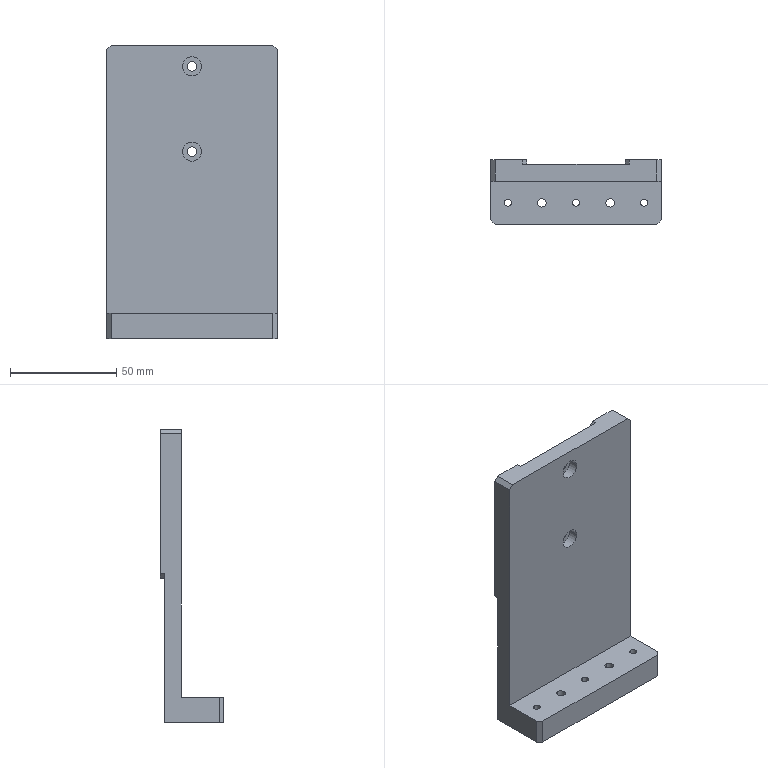Component | SolidWorks | 170423A4-PowerDockingCylinderFixingPlate-1 | 1 solid | 48 faces | box 80 x 30 x 138 mm | volume 110857 mm3 | plane 26 | cylinder 18 | cone 4 | commonest cylinder face diameters 3.3 x6 4 x4 9 x4 4.5 x4
build123d program:
from build123d import *

# Parameters (mm, degrees)
SKETCH1_W                                       = 80
SKETCH1_H                                       = 138
BOSS_EXTRUDE1_DEPTH                             = 8
SKETCH3_W                                       = 80
SKETCH3_H                                       = 12
BOSS_EXTRUDE2_DEPTH                             = 20
SKETCH4_W                                       = 16.95
SKETCH4_H                                       = 70
BOSS_EXTRUDE3_DEPTH                             = 2
CHAMFER1_SIZE                                   = 2
M4_TAPPED_HOLE1_D                               = 3.3
M4_HEX_SOCKET_HEAD_CAP_SCREW_CBORE1_D           = 4.5
M4_HEX_SOCKET_HEAD_CAP_SCREW_CBORE1_CBORE_D     = 9
M4_HEX_SOCKET_HEAD_CAP_SCREW_CBORE1_CBORE_DEPTH = 4.5
F_4_0_4_DIAMETER_HOLE1_D                        = 4
CHAMFER2_SIZE                                   = 0.5


with BuildPart() as part:
    # Sketch1 → Boss-Extrude1 (new body)
    with BuildSketch(Plane.XY):
        with Locations((0, 69)):
            Rectangle(SKETCH1_W, SKETCH1_H)
    extrude(amount=BOSS_EXTRUDE1_DEPTH)

    # Sketch3 → Boss-Extrude2 (add)
    with BuildSketch(Plane.XY.offset(8)):
        with Locations((0, 6)):
            Rectangle(SKETCH3_W, SKETCH3_H)
    extrude(amount=BOSS_EXTRUDE2_DEPTH)

    # Sketch4 → Boss-Extrude3 (add)
    with BuildSketch(Plane(origin=(0, 0, 0), x_dir=(-1, 0, 0), z_dir=(0, 0, -1))):
        with Locations((31.525, 103)):
            Rectangle(SKETCH4_W, SKETCH4_H)
        with Locations((-31.525, 103)):
            Rectangle(SKETCH4_W, SKETCH4_H)
    extrude(amount=BOSS_EXTRUDE3_DEPTH)

    # Chamfer1
    chamfer1_edges = [part.edges().sort_by_distance(p)[0] for p in [
        (40, 6, 28),
        (-40, 6, 28),
        (-40, 68, -1),
        (-23.05, 138, -1),
        (-23.05, 68, -1),
        (40, 68, -1),
        (23.05, 68, -1),
        (23.05, 138, -1),
        (-40, 138, 3),
        (40, 138, 3),
    ]]
    chamfer(chamfer1_edges, length=CHAMFER1_SIZE)

    # M4 Tapped Hole1 (through all)
    with Locations(Plane(origin=(0, 12, 0), x_dir=(1, 0, 0), z_dir=(0, 1, 0))):
        with Locations((32, -18), (0, -18), (-32, -18)):
            Hole(M4_TAPPED_HOLE1_D / 2)

    # M4 Hex Socket Head Cap Screw CBORE1 (through all)
    with Locations(Plane.XY.offset(8)):
        with Locations((0, 128), (0, 88)):
            CounterBoreHole(M4_HEX_SOCKET_HEAD_CAP_SCREW_CBORE1_D / 2, M4_HEX_SOCKET_HEAD_CAP_SCREW_CBORE1_CBORE_D / 2, M4_HEX_SOCKET_HEAD_CAP_SCREW_CBORE1_CBORE_DEPTH)

    # 4.0 _4_ Diameter Hole1 (through all)
    with Locations(Plane(origin=(0, 0, 0), x_dir=(-1, 0, 0), z_dir=(0, -1, 0))):
        with Locations((16, -18), (-16, -18)):
            Hole(F_4_0_4_DIAMETER_HOLE1_D / 2)

    # Chamfer2
    chamfer2_edges = [part.edges().sort_by_distance(p)[0] for p in [
        (-18, 0, 18),
        (14, 0, 18),
    ]]
    chamfer(chamfer2_edges, length=CHAMFER2_SIZE)


solid = part.part

# Placed as in the assembly
solid = solid.moved(Location((28.687, -57.611, -44.074), (90, 0, 0)))